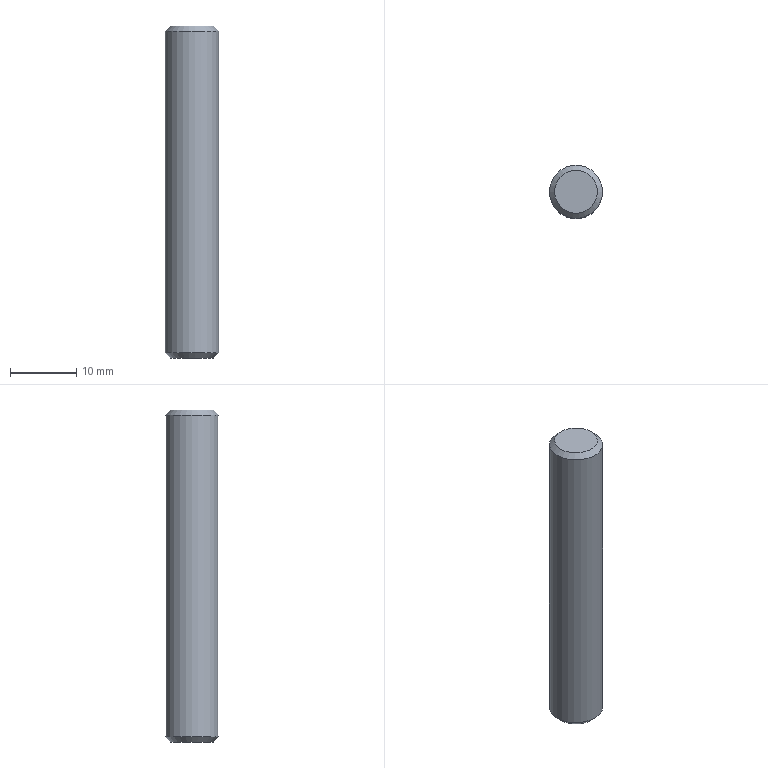Component | NX | 12_STUD_2 | 1 solid | 5 faces | volume 2499 mm3 | plane 2 | cone 2 | cylinder 1 | commonest cylinder face diameters 8 x1